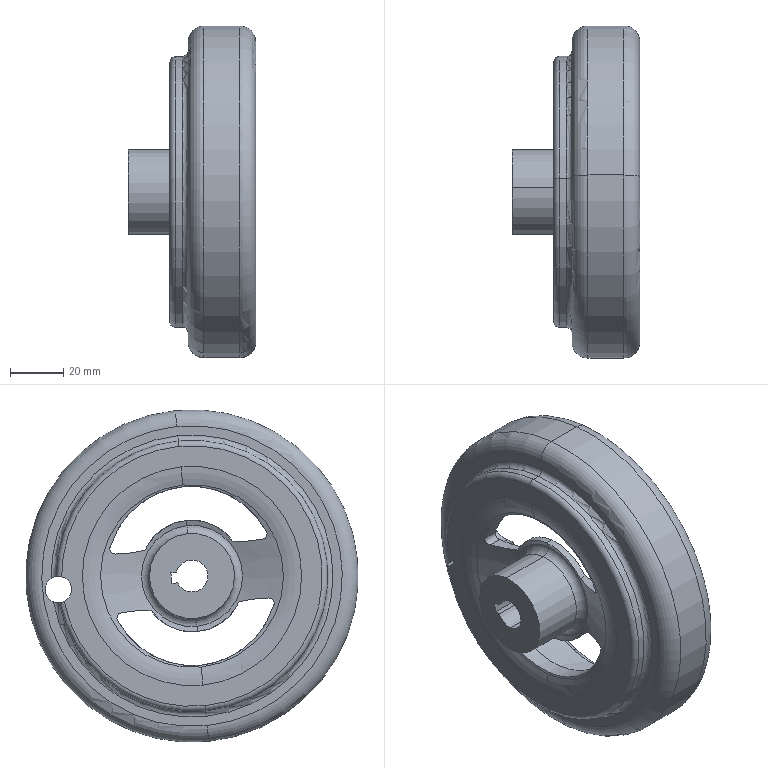Component | SolidWorks | PHSLN125-1_PHSLN125_1_1-1 | 1 solid | 71 faces | volume 196126 mm3 | cylinder 31 | torus 24 | plane 10 | cone 6 | commonest cylinder face diameters 100 x6 4 x4 12 x3 18.5 x3 38.4 x3 63.8 x3 102 x3 10 x2 | material '-